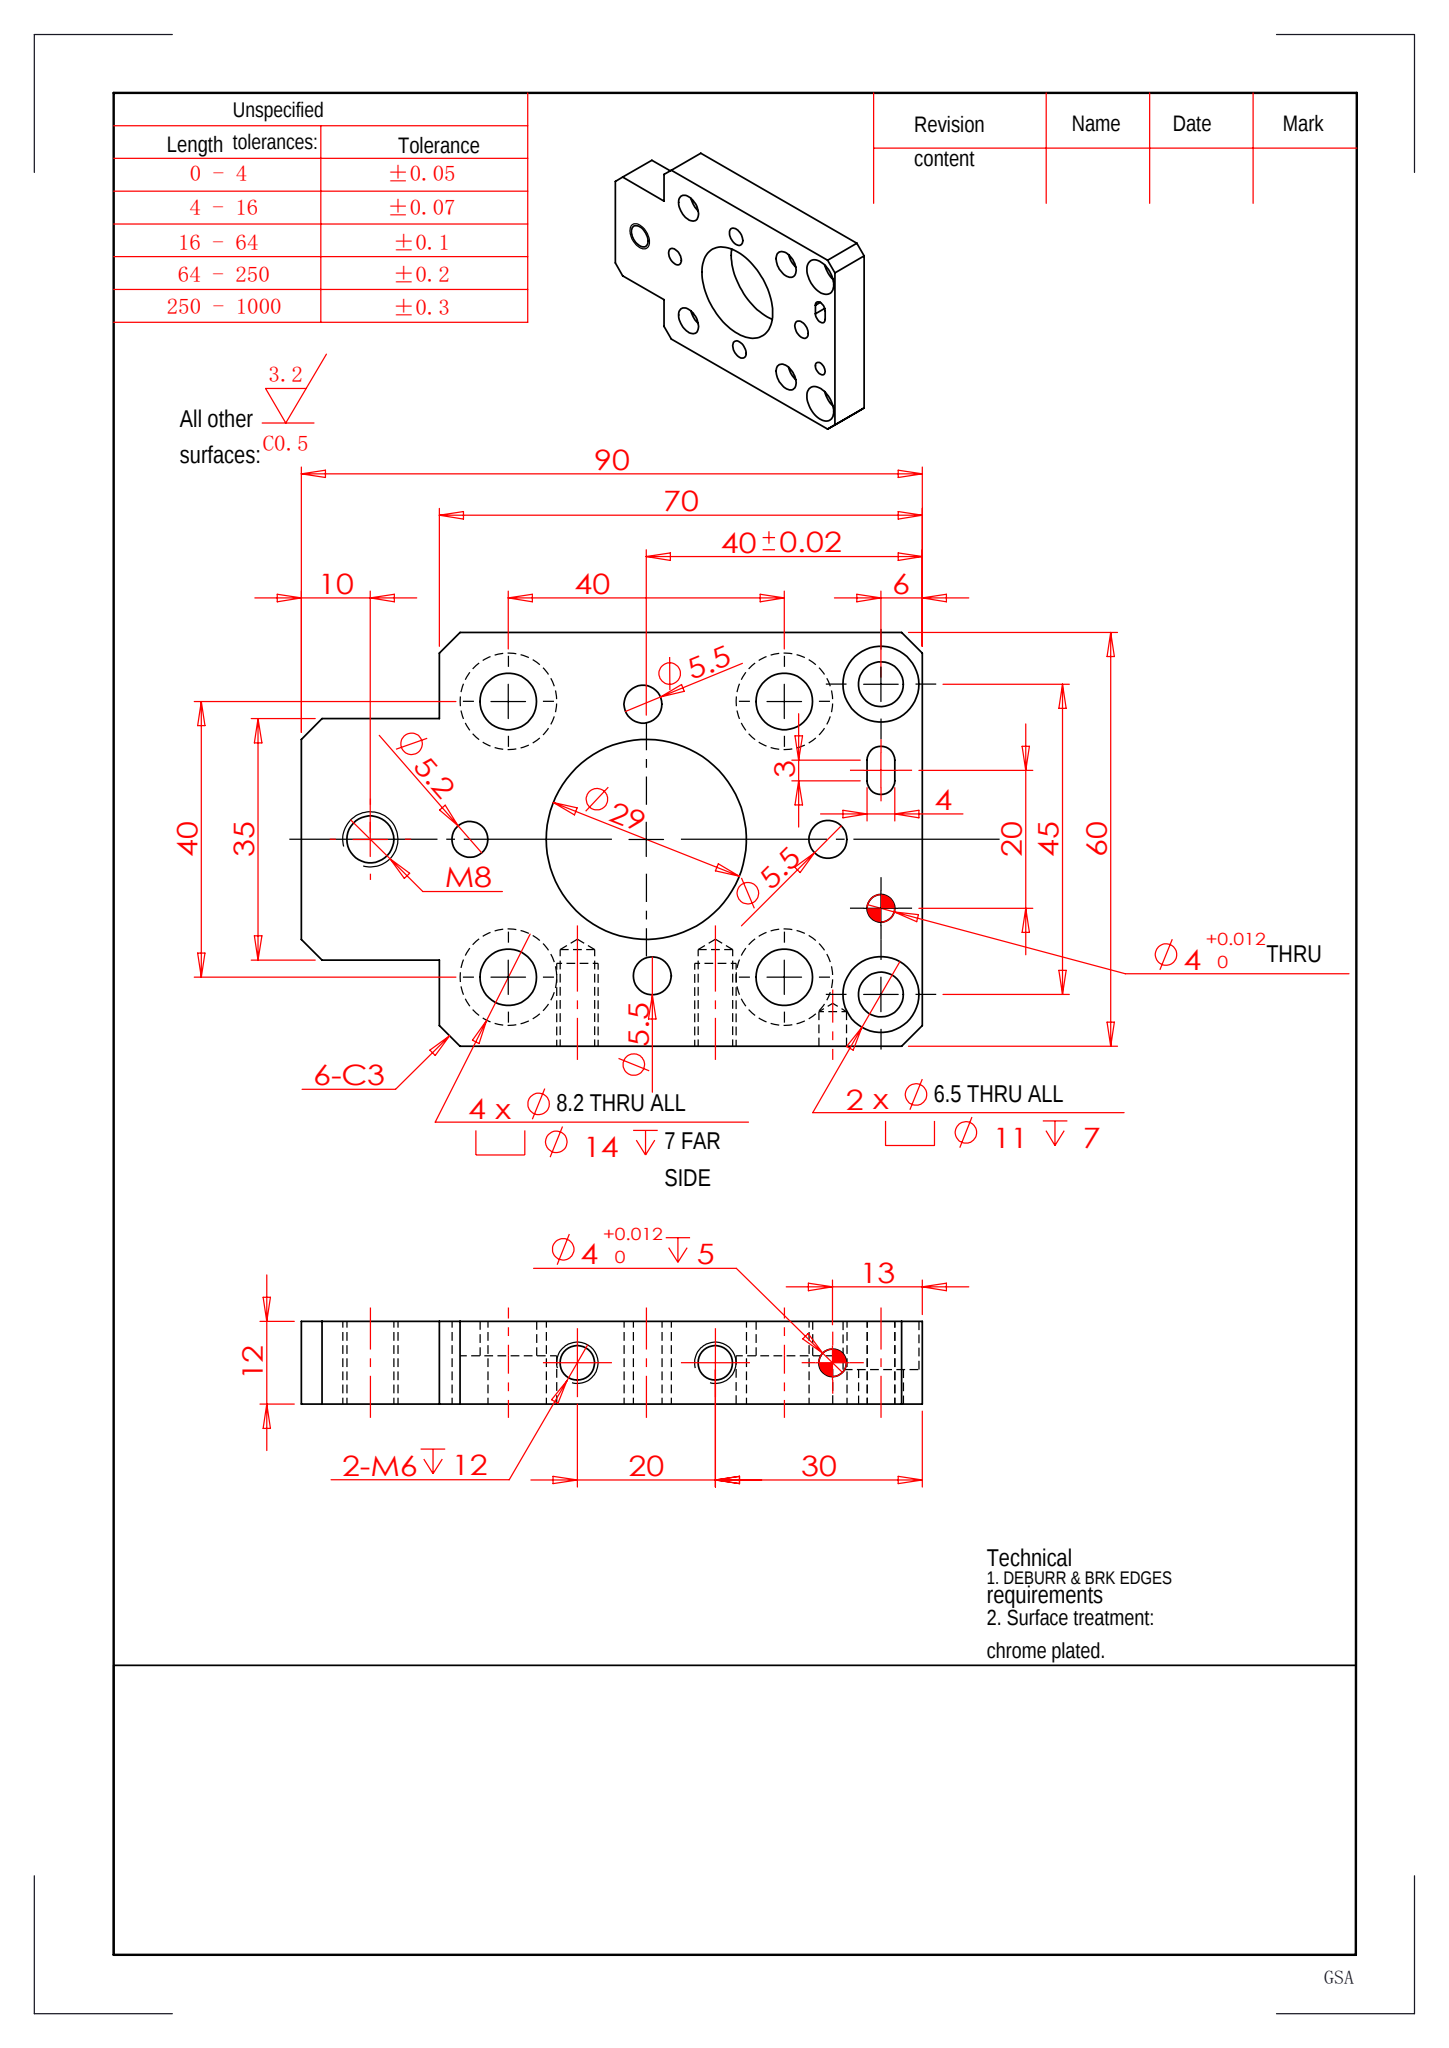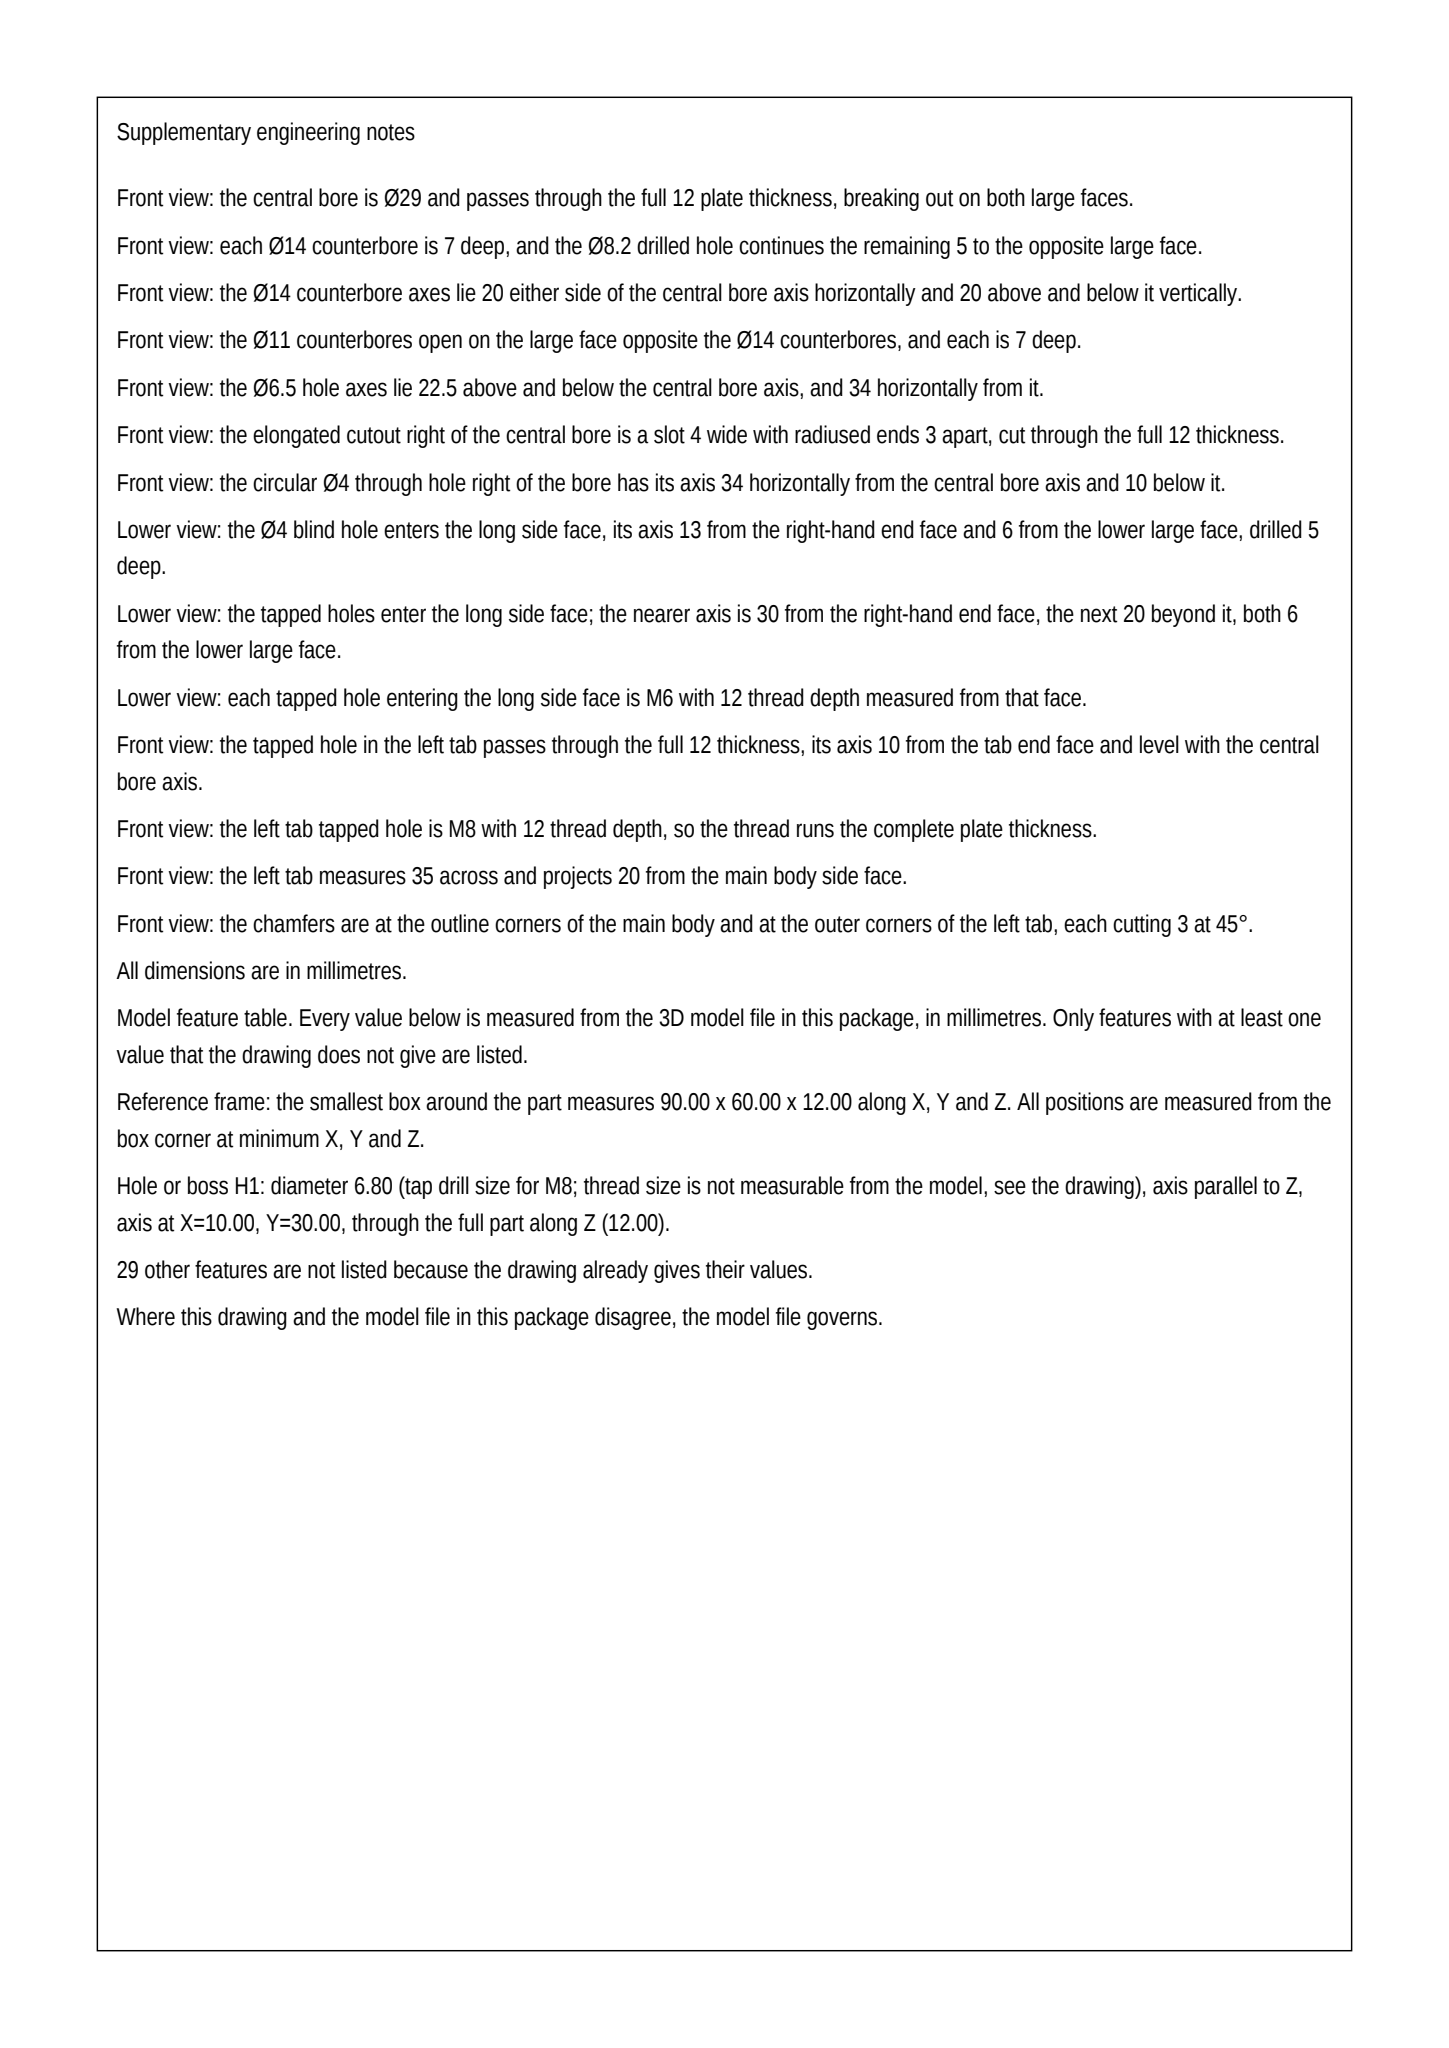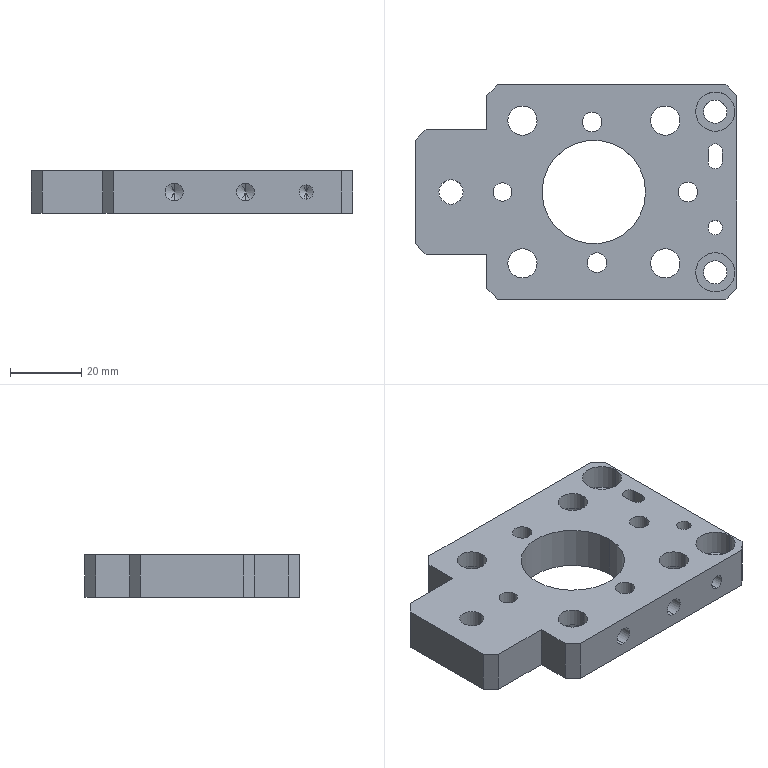Part | SolidWorks | mm | 1 solid | 76 faces | box 90 x 60 x 12 mm | volume 40892 mm3 | cylinder 46 | plane 24 | cone 6 | commonest cylinder face diameters 14 x8 8.2 x8 5.5 x6 4 x6 5 x4 11 x4 6.5 x4 5.2 x2
Drawing notes:
Ø5.2 THRU: 24.44 FROM LEFT EDGE, ON HORIZ CL (30 FROM BTM) | from the solid: cyl dia 5.2 axis z at (24.44, 30.0), len 12 thru
Ø5.5 THRU RH: 76.32 FROM LEFT EDGE, ON HORIZ CL (30 FROM BTM) | from the solid: cyl dia 5.5 axis z at (76.32, 30.0), len 12 thru
Ø5.5 THRU UPR: 49.52 FROM LEFT EDGE, 49.6 FROM BTM EDGE | from the solid: cyl dia 5.5 axis z at (49.52, 49.6), len 12 thru
Ø5.5 THRU LWR: 50.86 FROM LEFT EDGE, 10.21 FROM BTM EDGE | from the solid: cyl dia 5.5 axis z at (50.86, 10.21), len 12 thru
build123d program:
from build123d import *

# Parameters (mm, degrees)
SKETCH1_W                                            = 70
SKETCH1_H                                            = 60
BOSS_EXTRUDE1_DEPTH                                  = 12
SKETCH2_R                                            = 14.5
CUT_EXTRUDE1_DEPTH                                   = 48.634
HOLE_SIZE_ACCORDING_TO_HEX_SOCKET_HEAD_C_D           = 8.2
HOLE_SIZE_ACCORDING_TO_HEX_SOCKET_HEAD_C_CBORE_D     = 14
HOLE_SIZE_ACCORDING_TO_HEX_SOCKET_HEAD_C_CBORE_DEPTH = 7
CHAMFER2_SIZE                                        = 3
HOLE_SIZE_ACCORDING_TO_HEX_SOCKET_HE_2_D             = 6.5
HOLE_SIZE_ACCORDING_TO_HEX_SOCKET_HE_2_CBORE_D       = 11
HOLE_SIZE_ACCORDING_TO_HEX_SOCKET_HE_2_CBORE_DEPTH   = 7
SKETCH5_R                                            = 2
CUT_EXTRUDE2_DEPTH                                   = 48.634
M6_TAPPED_HOLE1_D                                    = 5
M6_TAPPED_HOLE1_DEPTH                                = 14
M6_TAPPED_HOLE1_TIP                                  = 1.502
SKETCH12_W                                           = 20
SKETCH12_H                                           = 35
BOSS_EXTRUDE2_DEPTH                                  = 12
CHAMFER3_SIZE                                        = 3
M8_TAPPED_HOLE1_D                                    = 6.8
F_4_0_4_DIAMETER_HOLE1_D                             = 4
F_4_0_4_DIAMETER_HOLE1_DEPTH                         = 5
F_4_0_4_DIAMETER_HOLE1_TIP                           = 1.202
SKETCH16_R                                           = 2.6
SKETCH16_R_2                                         = 2.75
CUT_EXTRUDE3_DEPTH                                   = 31


with BuildPart() as part:
    # Sketch1 → Boss-Extrude1 (new body)
    with BuildSketch(Plane.XY):
        Rectangle(SKETCH1_W, SKETCH1_H)
    extrude(amount=BOSS_EXTRUDE1_DEPTH)

    # Sketch2 → Cut-Extrude1 (cut, through all)
    with BuildSketch(Plane(origin=(0, 0, 0), x_dir=(-1, 0, 0), z_dir=(0, 0, -1))):
        with Locations((5, 0)):
            Circle(SKETCH2_R)
    extrude(amount=-CUT_EXTRUDE1_DEPTH, mode=Mode.SUBTRACT)

    # Hole Size according to Hex Socket Head C (through all)
    with Locations(Plane(origin=(15, 20, 0), x_dir=(-1, 0, 0), z_dir=(0, 0, -1))):
        with Locations((0, 0), (40, 0), (40, -40), (0, -40)):
            CounterBoreHole(HOLE_SIZE_ACCORDING_TO_HEX_SOCKET_HEAD_C_D / 2, HOLE_SIZE_ACCORDING_TO_HEX_SOCKET_HEAD_C_CBORE_D / 2, HOLE_SIZE_ACCORDING_TO_HEX_SOCKET_HEAD_C_CBORE_DEPTH)

    # Chamfer2
    chamfer2_edges = [part.edges().sort_by_distance(p)[0] for p in [
        (35, -30, 6),
        (-35, -30, 6),
        (-35, 30, 6),
        (35, 30, 6),
    ]]
    chamfer(chamfer2_edges, length=CHAMFER2_SIZE)

    # Hole Size according to Hex Socket He 2 (through all)
    with Locations(Plane(origin=(29, -22.5, 12), x_dir=(1, 0, 0), z_dir=(0, 0, 1))):
        with Locations((0, 0), (0, 45)):
            CounterBoreHole(HOLE_SIZE_ACCORDING_TO_HEX_SOCKET_HE_2_D / 2, HOLE_SIZE_ACCORDING_TO_HEX_SOCKET_HE_2_CBORE_D / 2, HOLE_SIZE_ACCORDING_TO_HEX_SOCKET_HE_2_CBORE_DEPTH)

    # Sketch5 → Cut-Extrude2 (cut, through all)
    with BuildSketch(Plane(origin=(0, 0, 12), x_dir=(-1, 0, 0), z_dir=(0, 0, -1))):
        with Locations((-29, -10)):
            Circle(SKETCH5_R)
        with BuildLine():
            Line((-31, 8.5), (-31, 11.5))
            ThreePointArc((-31, 11.5), (-29, 13.5), (-27, 11.5))
            Line((-27, 11.5), (-27, 8.5))
            ThreePointArc((-27, 8.5), (-29, 6.5), (-31, 8.5))
        make_face()
    extrude(amount=CUT_EXTRUDE2_DEPTH, mode=Mode.SUBTRACT)

    # M6 Tapped Hole1
    with Locations(Plane(origin=(-15, -30, 6), x_dir=(0, 0, -1), z_dir=(0, -1, 0))):
        with Locations((0, 0), (0, 20)):
            Hole(M6_TAPPED_HOLE1_D / 2, depth=M6_TAPPED_HOLE1_DEPTH)
            with Locations((0, 0, -(M6_TAPPED_HOLE1_DEPTH + M6_TAPPED_HOLE1_TIP / 2))):  # 118° drill point
                Cone(0, M6_TAPPED_HOLE1_D / 2, M6_TAPPED_HOLE1_TIP, mode=Mode.SUBTRACT)

    # Sketch12 → Boss-Extrude2 (add)
    with BuildSketch(Plane.XY.offset(12)):
        with Locations((-45, 0)):
            Rectangle(SKETCH12_W, SKETCH12_H)
    extrude(amount=-BOSS_EXTRUDE2_DEPTH)

    # Chamfer3
    chamfer3_edges = [part.edges().sort_by_distance(p)[0] for p in [
        (-55, 17.5, 6),
        (-55, -17.5, 6),
    ]]
    chamfer(chamfer3_edges, length=CHAMFER3_SIZE)

    # M8 Tapped Hole1 (through all)
    with Locations(Plane.XY.offset(12)):
        with Locations((-45, 0)):
            Hole(M8_TAPPED_HOLE1_D / 2)

    # 4.0 _4_ Diameter Hole1
    with Locations(Plane(origin=(22, -30, 6), x_dir=(0, 0, -1), z_dir=(0, -1, 0))):
        with Locations((0, 0)):
            Hole(F_4_0_4_DIAMETER_HOLE1_D / 2, depth=F_4_0_4_DIAMETER_HOLE1_DEPTH)
            with Locations((0, 0, -(F_4_0_4_DIAMETER_HOLE1_DEPTH + F_4_0_4_DIAMETER_HOLE1_TIP / 2))):  # 118° drill point
                Cone(0, F_4_0_4_DIAMETER_HOLE1_D / 2, F_4_0_4_DIAMETER_HOLE1_TIP, mode=Mode.SUBTRACT)

    # Sketch16 → Cut-Extrude3 (cut)
    with BuildSketch(Plane.XY.offset(12)):
        with Locations((-30.562, 0)):
            Circle(SKETCH16_R)
        with Locations((21.323, 0)):
            Circle(SKETCH16_R_2)
        with Locations((-5.484, 19.601)):
            Circle(SKETCH16_R_2)
        with Locations((-4.139, -19.793)):
            Circle(SKETCH16_R_2)
    extrude(amount=-CUT_EXTRUDE3_DEPTH, mode=Mode.SUBTRACT)


solid = part.part